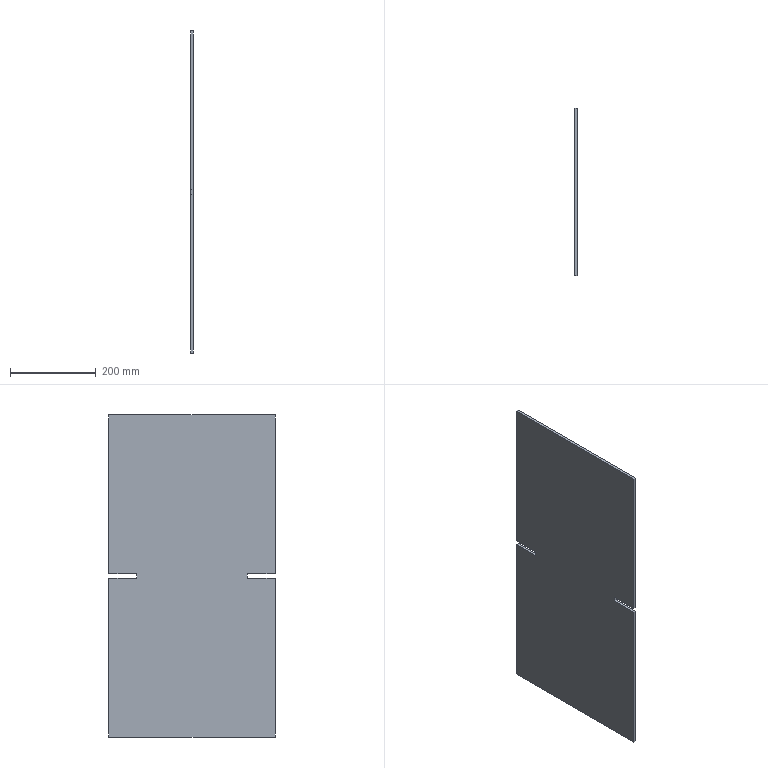Component | SolidWorks | Main-1_750X388X6-10 | 1 solid | 14 faces | box 6 x 388 x 750 mm | volume 1738200 mm3 | plane 14 | material Plain Carbon Steel
STEP:
#1=COLOUR_RGB('',0.7922,0.8196,0.9333);
#2=FILL_AREA_STYLE_COLOUR('',#1);
#3=FILL_AREA_STYLE('',(#2));
#4=SURFACE_STYLE_FILL_AREA(#3);
#5=SURFACE_SIDE_STYLE('',(#4));
#6=SURFACE_STYLE_USAGE(.BOTH.,#5);
#7=PRESENTATION_STYLE_ASSIGNMENT((#6));
#8=CARTESIAN_POINT('',(88.969,83.28,219.133));
#9=VERTEX_POINT('',#8);
#10=CARTESIAN_POINT('',(88.969,83.28,204.566));
#11=VERTEX_POINT('',#10);
#12=CARTESIAN_POINT('',(88.969,83.28,204.566));
#13=DIRECTION('',(0.,0.,-1.));
#14=VECTOR('',#13,39.37);
#15=LINE('',#12,#14);
#16=EDGE_CURVE('',#9,#11,#15,.T.);
#17=ORIENTED_EDGE('',*,*,#16,.F.);
#18=CARTESIAN_POINT('',(89.205,83.28,219.133));
#19=VERTEX_POINT('',#18);
#20=CARTESIAN_POINT('',(89.205,83.28,219.133));
#21=DIRECTION('',(-1.,0.,0.));
#22=VECTOR('',#21,39.37);
#23=LINE('',#20,#22);
#24=EDGE_CURVE('',#19,#9,#23,.T.);
#25=ORIENTED_EDGE('',*,*,#24,.F.);
#26=CARTESIAN_POINT('',(89.205,83.28,204.566));
#27=VERTEX_POINT('',#26);
#28=CARTESIAN_POINT('',(89.205,83.28,204.566));
#29=DIRECTION('',(0.,0.,-1.));
#30=VECTOR('',#29,39.37);
#31=LINE('',#28,#30);
#32=EDGE_CURVE('',#19,#27,#31,.T.);
#33=ORIENTED_EDGE('',*,*,#32,.T.);
#34=CARTESIAN_POINT('',(89.205,83.28,204.566));
#35=DIRECTION('',(-1.,0.,0.));
#36=VECTOR('',#35,39.37);
#37=LINE('',#34,#36);
#38=EDGE_CURVE('',#27,#11,#37,.T.);
#39=ORIENTED_EDGE('',*,*,#38,.T.);
#40=EDGE_LOOP('',(#17,#25,#33,#39));
#41=FACE_OUTER_BOUND('',#40,.T.);
#42=CARTESIAN_POINT('',(89.205,83.28,204.566));
#43=DIRECTION('',(0.,1.,0.));
#44=DIRECTION('',(0.,0.,-1.));
#45=AXIS2_PLACEMENT_3D('',#42,#43,#44);
#46=PLANE('',#45);
#47=ADVANCED_FACE('',(#41),#46,.T.);
#48=CARTESIAN_POINT('',(88.969,68.005,219.133));
#49=VERTEX_POINT('',#48);
#50=CARTESIAN_POINT('',(88.969,83.28,219.133));
#51=DIRECTION('',(0.,1.,0.));
#52=VECTOR('',#51,39.37);
#53=LINE('',#50,#52);
#54=EDGE_CURVE('',#49,#9,#53,.T.);
#55=ORIENTED_EDGE('',*,*,#54,.F.);
#56=CARTESIAN_POINT('',(89.205,68.005,219.133));
#57=VERTEX_POINT('',#56);
#58=CARTESIAN_POINT('',(89.205,68.005,219.133));
#59=DIRECTION('',(-1.,0.,0.));
#60=VECTOR('',#59,39.37);
#61=LINE('',#58,#60);
#62=EDGE_CURVE('',#57,#49,#61,.T.);
#63=ORIENTED_EDGE('',*,*,#62,.F.);
#64=CARTESIAN_POINT('',(89.205,83.28,219.133));
#65=DIRECTION('',(0.,1.,0.));
#66=VECTOR('',#65,39.37);
#67=LINE('',#64,#66);
#68=EDGE_CURVE('',#57,#19,#67,.T.);
#69=ORIENTED_EDGE('',*,*,#68,.T.);
#70=ORIENTED_EDGE('',*,*,#24,.T.);
#71=EDGE_LOOP('',(#55,#63,#69,#70));
#72=FACE_OUTER_BOUND('',#71,.T.);
#73=CARTESIAN_POINT('',(89.205,83.28,219.133));
#74=DIRECTION('',(0.,-0.,1.));
#75=DIRECTION('',(0.,1.,0.));
#76=AXIS2_PLACEMENT_3D('',#73,#74,#75);
#77=PLANE('',#76);
#78=ADVANCED_FACE('',(#72),#77,.T.);
#79=CARTESIAN_POINT('',(88.969,68.005,204.566));
#80=VERTEX_POINT('',#79);
#81=CARTESIAN_POINT('',(88.969,68.005,219.133));
#82=DIRECTION('',(0.,-0.,1.));
#83=VECTOR('',#82,39.37);
#84=LINE('',#81,#83);
#85=EDGE_CURVE('',#80,#49,#84,.T.);
#86=ORIENTED_EDGE('',*,*,#85,.F.);
#87=CARTESIAN_POINT('',(89.205,68.005,204.566));
#88=VERTEX_POINT('',#87);
#89=CARTESIAN_POINT('',(89.205,68.005,204.566));
#90=DIRECTION('',(-1.,0.,0.));
#91=VECTOR('',#90,39.37);
#92=LINE('',#89,#91);
#93=EDGE_CURVE('',#88,#80,#92,.T.);
#94=ORIENTED_EDGE('',*,*,#93,.F.);
#95=CARTESIAN_POINT('',(89.205,68.005,219.133));
#96=DIRECTION('',(0.,-0.,1.));
#97=VECTOR('',#96,39.37);
#98=LINE('',#95,#97);
#99=EDGE_CURVE('',#88,#57,#98,.T.);
#100=ORIENTED_EDGE('',*,*,#99,.T.);
#101=ORIENTED_EDGE('',*,*,#62,.T.);
#102=EDGE_LOOP('',(#86,#94,#100,#101));
#103=FACE_OUTER_BOUND('',#102,.T.);
#104=CARTESIAN_POINT('',(89.205,68.005,219.133));
#105=DIRECTION('',(-0.,-1.,-0.));
#106=DIRECTION('',(0.,-0.,1.));
#107=AXIS2_PLACEMENT_3D('',#104,#105,#106);
#108=PLANE('',#107);
#109=ADVANCED_FACE('',(#103),#108,.T.);
#110=CARTESIAN_POINT('',(88.969,70.564,204.566));
#111=VERTEX_POINT('',#110);
#112=CARTESIAN_POINT('',(88.969,68.005,204.566));
#113=DIRECTION('',(-0.,-1.,-0.));
#114=VECTOR('',#113,39.37);
#115=LINE('',#112,#114);
#116=EDGE_CURVE('',#111,#80,#115,.T.);
#117=ORIENTED_EDGE('',*,*,#116,.F.);
#118=CARTESIAN_POINT('',(89.205,70.564,204.566));
#119=VERTEX_POINT('',#118);
#120=CARTESIAN_POINT('',(89.205,70.564,204.566));
#121=DIRECTION('',(-1.,0.,0.));
#122=VECTOR('',#121,39.37);
#123=LINE('',#120,#122);
#124=EDGE_CURVE('',#119,#111,#123,.T.);
#125=ORIENTED_EDGE('',*,*,#124,.F.);
#126=CARTESIAN_POINT('',(89.205,68.005,204.566));
#127=DIRECTION('',(-0.,-1.,-0.));
#128=VECTOR('',#127,39.37);
#129=LINE('',#126,#128);
#130=EDGE_CURVE('',#119,#88,#129,.T.);
#131=ORIENTED_EDGE('',*,*,#130,.T.);
#132=ORIENTED_EDGE('',*,*,#93,.T.);
#133=EDGE_LOOP('',(#117,#125,#131,#132));
#134=FACE_OUTER_BOUND('',#133,.T.);
#135=CARTESIAN_POINT('',(89.205,68.005,204.566));
#136=DIRECTION('',(-0.,0.,-1.));
#137=DIRECTION('',(-0.,-1.,-0.));
#138=AXIS2_PLACEMENT_3D('',#135,#136,#137);
#139=PLANE('',#138);
#140=ADVANCED_FACE('',(#134),#139,.T.);
#141=CARTESIAN_POINT('',(88.969,70.564,204.172));
#142=VERTEX_POINT('',#141);
#143=CARTESIAN_POINT('',(88.969,70.564,204.566));
#144=DIRECTION('',(0.,-0.,1.));
#145=VECTOR('',#144,39.37);
#146=LINE('',#143,#145);
#147=EDGE_CURVE('',#142,#111,#146,.T.);
#148=ORIENTED_EDGE('',*,*,#147,.F.);
#149=CARTESIAN_POINT('',(89.205,70.564,204.172));
#150=VERTEX_POINT('',#149);
#151=CARTESIAN_POINT('',(89.205,70.564,204.172));
#152=DIRECTION('',(-1.,0.,0.));
#153=VECTOR('',#152,39.37);
#154=LINE('',#151,#153);
#155=EDGE_CURVE('',#150,#142,#154,.T.);
#156=ORIENTED_EDGE('',*,*,#155,.F.);
#157=CARTESIAN_POINT('',(89.205,70.564,204.566));
#158=DIRECTION('',(0.,-0.,1.));
#159=VECTOR('',#158,39.37);
#160=LINE('',#157,#159);
#161=EDGE_CURVE('',#150,#119,#160,.T.);
#162=ORIENTED_EDGE('',*,*,#161,.T.);
#163=ORIENTED_EDGE('',*,*,#124,.T.);
#164=EDGE_LOOP('',(#148,#156,#162,#163));
#165=FACE_OUTER_BOUND('',#164,.T.);
#166=CARTESIAN_POINT('',(89.205,70.564,204.566));
#167=DIRECTION('',(-0.,-1.,-0.));
#168=DIRECTION('',(0.,-0.,1.));
#169=AXIS2_PLACEMENT_3D('',#166,#167,#168);
#170=PLANE('',#169);
#171=ADVANCED_FACE('',(#165),#170,.T.);
#172=CARTESIAN_POINT('',(88.969,68.005,204.172));
#173=VERTEX_POINT('',#172);
#174=CARTESIAN_POINT('',(88.969,70.564,204.172));
#175=DIRECTION('',(0.,1.,0.));
#176=VECTOR('',#175,39.37);
#177=LINE('',#174,#176);
#178=EDGE_CURVE('',#173,#142,#177,.T.);
#179=ORIENTED_EDGE('',*,*,#178,.F.);
#180=CARTESIAN_POINT('',(89.205,68.005,204.172));
#181=VERTEX_POINT('',#180);
#182=CARTESIAN_POINT('',(89.205,68.005,204.172));
#183=DIRECTION('',(-1.,0.,0.));
#184=VECTOR('',#183,39.37);
#185=LINE('',#182,#184);
#186=EDGE_CURVE('',#181,#173,#185,.T.);
#187=ORIENTED_EDGE('',*,*,#186,.F.);
#188=CARTESIAN_POINT('',(89.205,70.564,204.172));
#189=DIRECTION('',(0.,1.,0.));
#190=VECTOR('',#189,39.37);
#191=LINE('',#188,#190);
#192=EDGE_CURVE('',#181,#150,#191,.T.);
#193=ORIENTED_EDGE('',*,*,#192,.T.);
#194=ORIENTED_EDGE('',*,*,#155,.T.);
#195=EDGE_LOOP('',(#179,#187,#193,#194));
#196=FACE_OUTER_BOUND('',#195,.T.);
#197=CARTESIAN_POINT('',(89.205,70.564,204.172));
#198=DIRECTION('',(0.,-0.,1.));
#199=DIRECTION('',(0.,1.,0.));
#200=AXIS2_PLACEMENT_3D('',#197,#198,#199);
#201=PLANE('',#200);
#202=ADVANCED_FACE('',(#196),#201,.T.);
#203=CARTESIAN_POINT('',(88.969,68.005,189.605));
#204=VERTEX_POINT('',#203);
#205=CARTESIAN_POINT('',(88.969,68.005,204.172));
#206=DIRECTION('',(0.,-0.,1.));
#207=VECTOR('',#206,39.37);
#208=LINE('',#205,#207);
#209=EDGE_CURVE('',#204,#173,#208,.T.);
#210=ORIENTED_EDGE('',*,*,#209,.F.);
#211=CARTESIAN_POINT('',(89.205,68.005,189.605));
#212=VERTEX_POINT('',#211);
#213=CARTESIAN_POINT('',(89.205,68.005,189.605));
#214=DIRECTION('',(-1.,0.,0.));
#215=VECTOR('',#214,39.37);
#216=LINE('',#213,#215);
#217=EDGE_CURVE('',#212,#204,#216,.T.);
#218=ORIENTED_EDGE('',*,*,#217,.F.);
#219=CARTESIAN_POINT('',(89.205,68.005,204.172));
#220=DIRECTION('',(0.,-0.,1.));
#221=VECTOR('',#220,39.37);
#222=LINE('',#219,#221);
#223=EDGE_CURVE('',#212,#181,#222,.T.);
#224=ORIENTED_EDGE('',*,*,#223,.T.);
#225=ORIENTED_EDGE('',*,*,#186,.T.);
#226=EDGE_LOOP('',(#210,#218,#224,#225));
#227=FACE_OUTER_BOUND('',#226,.T.);
#228=CARTESIAN_POINT('',(89.205,68.005,204.172));
#229=DIRECTION('',(-0.,-1.,-0.));
#230=DIRECTION('',(0.,-0.,1.));
#231=AXIS2_PLACEMENT_3D('',#228,#229,#230);
#232=PLANE('',#231);
#233=ADVANCED_FACE('',(#227),#232,.T.);
#234=CARTESIAN_POINT('',(88.969,83.28,189.605));
#235=VERTEX_POINT('',#234);
#236=CARTESIAN_POINT('',(88.969,68.005,189.605));
#237=DIRECTION('',(-0.,-1.,-0.));
#238=VECTOR('',#237,39.37);
#239=LINE('',#236,#238);
#240=EDGE_CURVE('',#235,#204,#239,.T.);
#241=ORIENTED_EDGE('',*,*,#240,.F.);
#242=CARTESIAN_POINT('',(89.205,83.28,189.605));
#243=VERTEX_POINT('',#242);
#244=CARTESIAN_POINT('',(89.205,83.28,189.605));
#245=DIRECTION('',(-1.,0.,0.));
#246=VECTOR('',#245,39.37);
#247=LINE('',#244,#246);
#248=EDGE_CURVE('',#243,#235,#247,.T.);
#249=ORIENTED_EDGE('',*,*,#248,.F.);
#250=CARTESIAN_POINT('',(89.205,68.005,189.605));
#251=DIRECTION('',(-0.,-1.,-0.));
#252=VECTOR('',#251,39.37);
#253=LINE('',#250,#252);
#254=EDGE_CURVE('',#243,#212,#253,.T.);
#255=ORIENTED_EDGE('',*,*,#254,.T.);
#256=ORIENTED_EDGE('',*,*,#217,.T.);
#257=EDGE_LOOP('',(#241,#249,#255,#256));
#258=FACE_OUTER_BOUND('',#257,.T.);
#259=CARTESIAN_POINT('',(89.205,68.005,189.605));
#260=DIRECTION('',(-0.,0.,-1.));
#261=DIRECTION('',(-0.,-1.,-0.));
#262=AXIS2_PLACEMENT_3D('',#259,#260,#261);
#263=PLANE('',#262);
#264=ADVANCED_FACE('',(#258),#263,.T.);
#265=CARTESIAN_POINT('',(88.969,83.28,204.172));
#266=VERTEX_POINT('',#265);
#267=CARTESIAN_POINT('',(88.969,83.28,189.605));
#268=DIRECTION('',(0.,0.,-1.));
#269=VECTOR('',#268,39.37);
#270=LINE('',#267,#269);
#271=EDGE_CURVE('',#266,#235,#270,.T.);
#272=ORIENTED_EDGE('',*,*,#271,.F.);
#273=CARTESIAN_POINT('',(89.205,83.28,204.172));
#274=VERTEX_POINT('',#273);
#275=CARTESIAN_POINT('',(89.205,83.28,204.172));
#276=DIRECTION('',(-1.,0.,0.));
#277=VECTOR('',#276,39.37);
#278=LINE('',#275,#277);
#279=EDGE_CURVE('',#274,#266,#278,.T.);
#280=ORIENTED_EDGE('',*,*,#279,.F.);
#281=CARTESIAN_POINT('',(89.205,83.28,189.605));
#282=DIRECTION('',(0.,0.,-1.));
#283=VECTOR('',#282,39.37);
#284=LINE('',#281,#283);
#285=EDGE_CURVE('',#274,#243,#284,.T.);
#286=ORIENTED_EDGE('',*,*,#285,.T.);
#287=ORIENTED_EDGE('',*,*,#248,.T.);
#288=EDGE_LOOP('',(#272,#280,#286,#287));
#289=FACE_OUTER_BOUND('',#288,.T.);
#290=CARTESIAN_POINT('',(89.205,83.28,189.605));
#291=DIRECTION('',(0.,1.,0.));
#292=DIRECTION('',(0.,0.,-1.));
#293=AXIS2_PLACEMENT_3D('',#290,#291,#292);
#294=PLANE('',#293);
#295=ADVANCED_FACE('',(#289),#294,.T.);
#296=CARTESIAN_POINT('',(88.969,80.721,204.172));
#297=VERTEX_POINT('',#296);
#298=CARTESIAN_POINT('',(88.969,83.28,204.172));
#299=DIRECTION('',(0.,1.,0.));
#300=VECTOR('',#299,39.37);
#301=LINE('',#298,#300);
#302=EDGE_CURVE('',#297,#266,#301,.T.);
#303=ORIENTED_EDGE('',*,*,#302,.F.);
#304=CARTESIAN_POINT('',(89.205,80.721,204.172));
#305=VERTEX_POINT('',#304);
#306=CARTESIAN_POINT('',(89.205,80.721,204.172));
#307=DIRECTION('',(-1.,0.,0.));
#308=VECTOR('',#307,39.37);
#309=LINE('',#306,#308);
#310=EDGE_CURVE('',#305,#297,#309,.T.);
#311=ORIENTED_EDGE('',*,*,#310,.F.);
#312=CARTESIAN_POINT('',(89.205,83.28,204.172));
#313=DIRECTION('',(0.,1.,0.));
#314=VECTOR('',#313,39.37);
#315=LINE('',#312,#314);
#316=EDGE_CURVE('',#305,#274,#315,.T.);
#317=ORIENTED_EDGE('',*,*,#316,.T.);
#318=ORIENTED_EDGE('',*,*,#279,.T.);
#319=EDGE_LOOP('',(#303,#311,#317,#318));
#320=FACE_OUTER_BOUND('',#319,.T.);
#321=CARTESIAN_POINT('',(89.205,83.28,204.172));
#322=DIRECTION('',(0.,-0.,1.));
#323=DIRECTION('',(0.,1.,0.));
#324=AXIS2_PLACEMENT_3D('',#321,#322,#323);
#325=PLANE('',#324);
#326=ADVANCED_FACE('',(#320),#325,.T.);
#327=CARTESIAN_POINT('',(88.969,80.721,204.566));
#328=VERTEX_POINT('',#327);
#329=CARTESIAN_POINT('',(88.969,80.721,204.172));
#330=DIRECTION('',(0.,0.,-1.));
#331=VECTOR('',#330,39.37);
#332=LINE('',#329,#331);
#333=EDGE_CURVE('',#328,#297,#332,.T.);
#334=ORIENTED_EDGE('',*,*,#333,.F.);
#335=CARTESIAN_POINT('',(89.205,80.721,204.566));
#336=VERTEX_POINT('',#335);
#337=CARTESIAN_POINT('',(89.205,80.721,204.566));
#338=DIRECTION('',(-1.,0.,0.));
#339=VECTOR('',#338,39.37);
#340=LINE('',#337,#339);
#341=EDGE_CURVE('',#336,#328,#340,.T.);
#342=ORIENTED_EDGE('',*,*,#341,.F.);
#343=CARTESIAN_POINT('',(89.205,80.721,204.172));
#344=DIRECTION('',(0.,0.,-1.));
#345=VECTOR('',#344,39.37);
#346=LINE('',#343,#345);
#347=EDGE_CURVE('',#336,#305,#346,.T.);
#348=ORIENTED_EDGE('',*,*,#347,.T.);
#349=ORIENTED_EDGE('',*,*,#310,.T.);
#350=EDGE_LOOP('',(#334,#342,#348,#349));
#351=FACE_OUTER_BOUND('',#350,.T.);
#352=CARTESIAN_POINT('',(89.205,80.721,204.172));
#353=DIRECTION('',(0.,1.,0.));
#354=DIRECTION('',(0.,0.,-1.));
#355=AXIS2_PLACEMENT_3D('',#352,#353,#354);
#356=PLANE('',#355);
#357=ADVANCED_FACE('',(#351),#356,.T.);
#358=CARTESIAN_POINT('',(88.969,80.721,204.566));
#359=DIRECTION('',(-0.,-1.,-0.));
#360=VECTOR('',#359,39.37);
#361=LINE('',#358,#360);
#362=EDGE_CURVE('',#11,#328,#361,.T.);
#363=ORIENTED_EDGE('',*,*,#362,.F.);
#364=ORIENTED_EDGE('',*,*,#38,.F.);
#365=CARTESIAN_POINT('',(89.205,80.721,204.566));
#366=DIRECTION('',(-0.,-1.,-0.));
#367=VECTOR('',#366,39.37);
#368=LINE('',#365,#367);
#369=EDGE_CURVE('',#27,#336,#368,.T.);
#370=ORIENTED_EDGE('',*,*,#369,.T.);
#371=ORIENTED_EDGE('',*,*,#341,.T.);
#372=EDGE_LOOP('',(#363,#364,#370,#371));
#373=FACE_OUTER_BOUND('',#372,.T.);
#374=CARTESIAN_POINT('',(89.205,80.721,204.566));
#375=DIRECTION('',(-0.,0.,-1.));
#376=DIRECTION('',(-0.,-1.,-0.));
#377=AXIS2_PLACEMENT_3D('',#374,#375,#376);
#378=PLANE('',#377);
#379=ADVANCED_FACE('',(#373),#378,.T.);
#380=ORIENTED_EDGE('',*,*,#32,.F.);
#381=ORIENTED_EDGE('',*,*,#68,.F.);
#382=ORIENTED_EDGE('',*,*,#99,.F.);
#383=ORIENTED_EDGE('',*,*,#130,.F.);
#384=ORIENTED_EDGE('',*,*,#161,.F.);
#385=ORIENTED_EDGE('',*,*,#192,.F.);
#386=ORIENTED_EDGE('',*,*,#223,.F.);
#387=ORIENTED_EDGE('',*,*,#254,.F.);
#388=ORIENTED_EDGE('',*,*,#285,.F.);
#389=ORIENTED_EDGE('',*,*,#316,.F.);
#390=ORIENTED_EDGE('',*,*,#347,.F.);
#391=ORIENTED_EDGE('',*,*,#369,.F.);
#392=EDGE_LOOP('',(#380,#381,#382,#383,#384,#385,#386,#387,#388,#389,#390,#391));
#393=FACE_OUTER_BOUND('',#392,.T.);
#394=CARTESIAN_POINT('',(89.205,83.28,219.133));
#395=DIRECTION('',(1.,-0.,-0.));
#396=DIRECTION('',(0.,-0.,1.));
#397=AXIS2_PLACEMENT_3D('',#394,#395,#396);
#398=PLANE('',#397);
#399=ADVANCED_FACE('',(#393),#398,.T.);
#400=ORIENTED_EDGE('',*,*,#16,.T.);
#401=ORIENTED_EDGE('',*,*,#362,.T.);
#402=ORIENTED_EDGE('',*,*,#333,.T.);
#403=ORIENTED_EDGE('',*,*,#302,.T.);
#404=ORIENTED_EDGE('',*,*,#271,.T.);
#405=ORIENTED_EDGE('',*,*,#240,.T.);
#406=ORIENTED_EDGE('',*,*,#209,.T.);
#407=ORIENTED_EDGE('',*,*,#178,.T.);
#408=ORIENTED_EDGE('',*,*,#147,.T.);
#409=ORIENTED_EDGE('',*,*,#116,.T.);
#410=ORIENTED_EDGE('',*,*,#85,.T.);
#411=ORIENTED_EDGE('',*,*,#54,.T.);
#412=EDGE_LOOP('',(#400,#401,#402,#403,#404,#405,#406,#407,#408,#409,#410,#411));
#413=FACE_OUTER_BOUND('',#412,.T.);
#414=CARTESIAN_POINT('',(88.969,83.28,219.133));
#415=DIRECTION('',(1.,-0.,-0.));
#416=DIRECTION('',(0.,-0.,1.));
#417=AXIS2_PLACEMENT_3D('',#414,#415,#416);
#418=PLANE('',#417);
#419=ADVANCED_FACE('',(#413),#418,.F.);
#420=CLOSED_SHELL('',(#47,#78,#109,#140,#171,#202,#233,#264,#295,#326,#357,#379,#399,#419));
#421=MANIFOLD_SOLID_BREP('',#420);
#422=STYLED_ITEM('',(#7),#421);
#423=(LENGTH_UNIT()NAMED_UNIT(*)SI_UNIT($,.METRE.));
#424=LENGTH_MEASURE_WITH_UNIT(LENGTH_MEASURE(0.0254),#423);
#425=DIMENSIONAL_EXPONENTS(1.,0.,0.,0.,0.,0.,0.);
#426=(CONVERSION_BASED_UNIT('',#424)LENGTH_UNIT()NAMED_UNIT(#425));
#427=UNCERTAINTY_MEASURE_WITH_UNIT(LENGTH_MEASURE(0.00001),#426,'','');
#428=(NAMED_UNIT(*)PLANE_ANGLE_UNIT()SI_UNIT($,.RADIAN.));
#429=(NAMED_UNIT(*)SI_UNIT($,.STERADIAN.)SOLID_ANGLE_UNIT());
#430=(GEOMETRIC_REPRESENTATION_CONTEXT(3)GLOBAL_UNCERTAINTY_ASSIGNED_CONTEXT((#427))GLOBAL_UNIT_ASSIGNED_CONTEXT((#426,#428,#429))REPRESENTATION_CONTEXT('',''));
#431=MECHANICAL_DESIGN_GEOMETRIC_PRESENTATION_REPRESENTATION('',(#422),#430);
#432=CARTESIAN_POINT('',(0.,0.,0.));
#433=DIRECTION('',(0.,0.,1.));
#434=DIRECTION('',(1.,0.,0.));
#435=AXIS2_PLACEMENT_3D('',#432,#433,#434);
#436=(LENGTH_UNIT()NAMED_UNIT(*)SI_UNIT($,.METRE.));
#437=LENGTH_MEASURE_WITH_UNIT(LENGTH_MEASURE(0.0254),#436);
#438=DIMENSIONAL_EXPONENTS(1.,0.,0.,0.,0.,0.,0.);
#439=(CONVERSION_BASED_UNIT('',#437)LENGTH_UNIT()NAMED_UNIT(#438));
#440=UNCERTAINTY_MEASURE_WITH_UNIT(LENGTH_MEASURE(0.00001),#439,'','');
#441=(NAMED_UNIT(*)PLANE_ANGLE_UNIT()SI_UNIT($,.RADIAN.));
#442=(NAMED_UNIT(*)SI_UNIT($,.STERADIAN.)SOLID_ANGLE_UNIT());
#443=(GEOMETRIC_REPRESENTATION_CONTEXT(3)GLOBAL_UNCERTAINTY_ASSIGNED_CONTEXT((#440))GLOBAL_UNIT_ASSIGNED_CONTEXT((#439,#441,#442))REPRESENTATION_CONTEXT('',''));
#444=ADVANCED_BREP_SHAPE_REPRESENTATION('',(#421,#435),#443);
#445=PRESENTATION_LAYER_ASSIGNMENT('','',(#422));